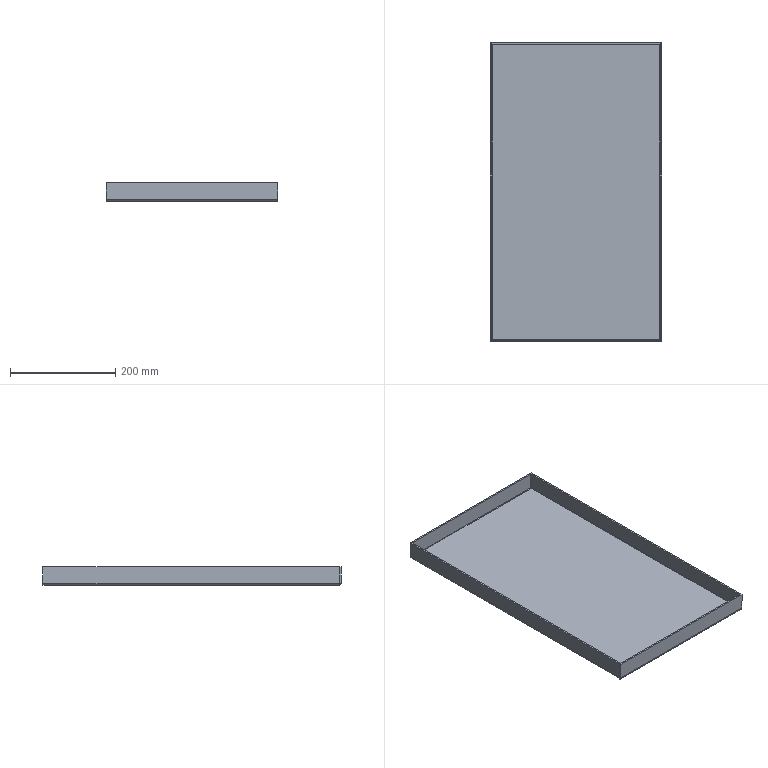Component | SolidWorks | MainBoardLowerBucklePlate-1 | 1 solid | 42 faces | box 326 x 566.5 x 35 mm | volume 718865 mm3 | plane 34 | cylinder 8 | commonest cylinder face diameters 7.473 x4 1.473 x4 | material Q235
STEP:
#1=CARTESIAN_POINT('',(-38.422,4.209,109.595));
#2=VERTEX_POINT('',#1);
#3=CARTESIAN_POINT('',(-38.422,4.206,109.595));
#4=VERTEX_POINT('',#3);
#5=CARTESIAN_POINT('',(-38.422,4.209,109.595));
#6=DIRECTION('',(-0.,-1.,-0.));
#7=VECTOR('',#6,39.37);
#8=LINE('',#5,#7);
#9=EDGE_CURVE('',#2,#4,#8,.T.);
#10=ORIENTED_EDGE('',*,*,#9,.T.);
#11=CARTESIAN_POINT('',(-38.422,4.062,109.477));
#12=VERTEX_POINT('',#11);
#13=CARTESIAN_POINT('',(-38.422,4.062,109.624));
#14=DIRECTION('',(-1.,-0.,0.));
#15=DIRECTION('',(0.,-0.,1.));
#16=AXIS2_PLACEMENT_3D('',#13,#14,#15);
#17=CIRCLE('',#16,0.1471);
#18=EDGE_CURVE('',#4,#12,#17,.T.);
#19=ORIENTED_EDGE('',*,*,#18,.T.);
#20=CARTESIAN_POINT('',(-38.422,4.209,109.477));
#21=VERTEX_POINT('',#20);
#22=CARTESIAN_POINT('',(-38.422,-17.947,109.477));
#23=DIRECTION('',(0.,-1.,-0.));
#24=VECTOR('',#23,39.37);
#25=LINE('',#22,#24);
#26=EDGE_CURVE('',#21,#12,#25,.T.);
#27=ORIENTED_EDGE('',*,*,#26,.F.);
#28=CARTESIAN_POINT('',(-38.422,4.209,109.595));
#29=DIRECTION('',(-0.,0.,-1.));
#30=VECTOR('',#29,39.37);
#31=LINE('',#28,#30);
#32=EDGE_CURVE('',#2,#21,#31,.T.);
#33=ORIENTED_EDGE('',*,*,#32,.F.);
#34=EDGE_LOOP('',(#10,#19,#27,#33));
#35=FACE_OUTER_BOUND('',#34,.T.);
#36=CARTESIAN_POINT('',(-38.422,4.209,109.595));
#37=DIRECTION('',(1.,-0.,-0.));
#38=DIRECTION('',(0.,1.,0.));
#39=AXIS2_PLACEMENT_3D('',#36,#37,#38);
#40=PLANE('',#39);
#41=ADVANCED_FACE('',(#35),#40,.T.);
#42=CARTESIAN_POINT('',(-25.882,4.209,109.477));
#43=VERTEX_POINT('',#42);
#44=CARTESIAN_POINT('',(-25.882,4.062,109.477));
#45=VERTEX_POINT('',#44);
#46=CARTESIAN_POINT('',(-25.882,4.209,109.477));
#47=DIRECTION('',(0.,-1.,-0.));
#48=VECTOR('',#47,39.37);
#49=LINE('',#46,#48);
#50=EDGE_CURVE('',#43,#45,#49,.T.);
#51=ORIENTED_EDGE('',*,*,#50,.T.);
#52=CARTESIAN_POINT('',(-25.882,4.206,109.595));
#53=VERTEX_POINT('',#52);
#54=CARTESIAN_POINT('',(-25.882,4.062,109.624));
#55=DIRECTION('',(1.,0.,-0.));
#56=DIRECTION('',(0.,0.,1.));
#57=AXIS2_PLACEMENT_3D('',#54,#55,#56);
#58=CIRCLE('',#57,0.1471);
#59=EDGE_CURVE('',#45,#53,#58,.T.);
#60=ORIENTED_EDGE('',*,*,#59,.T.);
#61=CARTESIAN_POINT('',(-25.882,4.209,109.595));
#62=VERTEX_POINT('',#61);
#63=CARTESIAN_POINT('',(-25.882,4.209,109.595));
#64=DIRECTION('',(0.,-1.,-0.));
#65=VECTOR('',#64,39.37);
#66=LINE('',#63,#65);
#67=EDGE_CURVE('',#62,#53,#66,.T.);
#68=ORIENTED_EDGE('',*,*,#67,.F.);
#69=CARTESIAN_POINT('',(-25.882,4.209,109.595));
#70=DIRECTION('',(-0.,0.,-1.));
#71=VECTOR('',#70,39.37);
#72=LINE('',#69,#71);
#73=EDGE_CURVE('',#62,#43,#72,.T.);
#74=ORIENTED_EDGE('',*,*,#73,.T.);
#75=EDGE_LOOP('',(#51,#60,#68,#74));
#76=FACE_OUTER_BOUND('',#75,.T.);
#77=CARTESIAN_POINT('',(-25.882,4.062,109.595));
#78=DIRECTION('',(-1.,0.,0.));
#79=DIRECTION('',(-0.,-1.,-0.));
#80=AXIS2_PLACEMENT_3D('',#77,#78,#79);
#81=PLANE('',#80);
#82=ADVANCED_FACE('',(#76),#81,.T.);
#83=CARTESIAN_POINT('',(-38.422,4.062,109.477));
#84=DIRECTION('',(1.,0.,-0.));
#85=VECTOR('',#84,39.37);
#86=LINE('',#83,#85);
#87=EDGE_CURVE('',#12,#45,#86,.T.);
#88=ORIENTED_EDGE('',*,*,#87,.T.);
#89=CARTESIAN_POINT('',(-25.882,-17.947,109.477));
#90=VERTEX_POINT('',#89);
#91=CARTESIAN_POINT('',(-25.882,4.209,109.477));
#92=DIRECTION('',(0.,-1.,-0.));
#93=VECTOR('',#92,39.37);
#94=LINE('',#91,#93);
#95=EDGE_CURVE('',#45,#90,#94,.T.);
#96=ORIENTED_EDGE('',*,*,#95,.T.);
#97=CARTESIAN_POINT('',(-38.422,-17.947,109.477));
#98=VERTEX_POINT('',#97);
#99=CARTESIAN_POINT('',(-25.734,-17.947,109.477));
#100=DIRECTION('',(-1.,-0.,0.));
#101=VECTOR('',#100,39.37);
#102=LINE('',#99,#101);
#103=EDGE_CURVE('',#90,#98,#102,.T.);
#104=ORIENTED_EDGE('',*,*,#103,.T.);
#105=CARTESIAN_POINT('',(-38.422,-17.947,109.477));
#106=DIRECTION('',(-0.,1.,0.));
#107=VECTOR('',#106,39.37);
#108=LINE('',#105,#107);
#109=EDGE_CURVE('',#98,#12,#108,.T.);
#110=ORIENTED_EDGE('',*,*,#109,.T.);
#111=EDGE_LOOP('',(#88,#96,#104,#110));
#112=FACE_OUTER_BOUND('',#111,.T.);
#113=CARTESIAN_POINT('',(-32.152,-6.942,109.477));
#114=DIRECTION('',(0.,-0.,1.));
#115=DIRECTION('',(-0.,1.,0.));
#116=AXIS2_PLACEMENT_3D('',#113,#114,#115);
#117=PLANE('',#116);
#118=ADVANCED_FACE('',(#112),#117,.F.);
#119=CARTESIAN_POINT('',(-25.882,4.062,109.595));
#120=VERTEX_POINT('',#119);
#121=CARTESIAN_POINT('',(-25.882,-17.947,109.595));
#122=VERTEX_POINT('',#121);
#123=CARTESIAN_POINT('',(-25.882,4.209,109.595));
#124=DIRECTION('',(0.,-1.,-0.));
#125=VECTOR('',#124,39.37);
#126=LINE('',#123,#125);
#127=EDGE_CURVE('',#120,#122,#126,.T.);
#128=ORIENTED_EDGE('',*,*,#127,.F.);
#129=CARTESIAN_POINT('',(-38.422,4.062,109.595));
#130=VERTEX_POINT('',#129);
#131=CARTESIAN_POINT('',(-38.422,4.062,109.595));
#132=DIRECTION('',(1.,0.,-0.));
#133=VECTOR('',#132,39.37);
#134=LINE('',#131,#133);
#135=EDGE_CURVE('',#130,#120,#134,.T.);
#136=ORIENTED_EDGE('',*,*,#135,.F.);
#137=CARTESIAN_POINT('',(-38.422,-17.947,109.595));
#138=VERTEX_POINT('',#137);
#139=CARTESIAN_POINT('',(-38.422,-17.947,109.595));
#140=DIRECTION('',(-0.,1.,0.));
#141=VECTOR('',#140,39.37);
#142=LINE('',#139,#141);
#143=EDGE_CURVE('',#138,#130,#142,.T.);
#144=ORIENTED_EDGE('',*,*,#143,.F.);
#145=CARTESIAN_POINT('',(-25.734,-17.947,109.595));
#146=DIRECTION('',(-1.,-0.,0.));
#147=VECTOR('',#146,39.37);
#148=LINE('',#145,#147);
#149=EDGE_CURVE('',#122,#138,#148,.T.);
#150=ORIENTED_EDGE('',*,*,#149,.F.);
#151=EDGE_LOOP('',(#128,#136,#144,#150));
#152=FACE_OUTER_BOUND('',#151,.T.);
#153=CARTESIAN_POINT('',(-32.152,-6.942,109.595));
#154=DIRECTION('',(0.,-0.,1.));
#155=DIRECTION('',(-0.,1.,0.));
#156=AXIS2_PLACEMENT_3D('',#153,#154,#155);
#157=PLANE('',#156);
#158=ADVANCED_FACE('',(#152),#157,.T.);
#159=CARTESIAN_POINT('',(-25.734,-17.947,109.477));
#160=VERTEX_POINT('',#159);
#161=CARTESIAN_POINT('',(-25.734,-17.947,109.477));
#162=DIRECTION('',(-1.,-0.,0.));
#163=VECTOR('',#162,39.37);
#164=LINE('',#161,#163);
#165=EDGE_CURVE('',#160,#90,#164,.T.);
#166=ORIENTED_EDGE('',*,*,#165,.T.);
#167=CARTESIAN_POINT('',(-25.737,-17.947,109.595));
#168=VERTEX_POINT('',#167);
#169=CARTESIAN_POINT('',(-25.882,-17.947,109.624));
#170=DIRECTION('',(0.,-1.,-0.));
#171=DIRECTION('',(0.,0.,-1.));
#172=AXIS2_PLACEMENT_3D('',#169,#170,#171);
#173=CIRCLE('',#172,0.1471);
#174=EDGE_CURVE('',#90,#168,#173,.T.);
#175=ORIENTED_EDGE('',*,*,#174,.T.);
#176=CARTESIAN_POINT('',(-25.734,-17.947,109.595));
#177=VERTEX_POINT('',#176);
#178=CARTESIAN_POINT('',(-25.734,-17.947,109.595));
#179=DIRECTION('',(-1.,-0.,0.));
#180=VECTOR('',#179,39.37);
#181=LINE('',#178,#180);
#182=EDGE_CURVE('',#177,#168,#181,.T.);
#183=ORIENTED_EDGE('',*,*,#182,.F.);
#184=CARTESIAN_POINT('',(-25.734,-17.947,109.595));
#185=DIRECTION('',(-0.,0.,-1.));
#186=VECTOR('',#185,39.37);
#187=LINE('',#184,#186);
#188=EDGE_CURVE('',#177,#160,#187,.T.);
#189=ORIENTED_EDGE('',*,*,#188,.T.);
#190=EDGE_LOOP('',(#166,#175,#183,#189));
#191=FACE_OUTER_BOUND('',#190,.T.);
#192=CARTESIAN_POINT('',(-25.882,-17.947,109.595));
#193=DIRECTION('',(-0.,1.,0.));
#194=DIRECTION('',(-0.,0.,-1.));
#195=AXIS2_PLACEMENT_3D('',#192,#193,#194);
#196=PLANE('',#195);
#197=ADVANCED_FACE('',(#191),#196,.T.);
#198=CARTESIAN_POINT('',(-38.569,-17.947,109.595));
#199=VERTEX_POINT('',#198);
#200=CARTESIAN_POINT('',(-38.566,-17.947,109.595));
#201=VERTEX_POINT('',#200);
#202=CARTESIAN_POINT('',(-38.569,-17.947,109.595));
#203=DIRECTION('',(1.,0.,0.));
#204=VECTOR('',#203,39.37);
#205=LINE('',#202,#204);
#206=EDGE_CURVE('',#199,#201,#205,.T.);
#207=ORIENTED_EDGE('',*,*,#206,.T.);
#208=CARTESIAN_POINT('',(-38.422,-17.947,109.624));
#209=DIRECTION('',(0.,-1.,-0.));
#210=DIRECTION('',(0.,0.,1.));
#211=AXIS2_PLACEMENT_3D('',#208,#209,#210);
#212=CIRCLE('',#211,0.1471);
#213=EDGE_CURVE('',#201,#98,#212,.T.);
#214=ORIENTED_EDGE('',*,*,#213,.T.);
#215=CARTESIAN_POINT('',(-38.569,-17.947,109.477));
#216=VERTEX_POINT('',#215);
#217=CARTESIAN_POINT('',(-25.734,-17.947,109.477));
#218=DIRECTION('',(1.,0.,-0.));
#219=VECTOR('',#218,39.37);
#220=LINE('',#217,#219);
#221=EDGE_CURVE('',#216,#98,#220,.T.);
#222=ORIENTED_EDGE('',*,*,#221,.F.);
#223=CARTESIAN_POINT('',(-38.569,-17.947,109.595));
#224=DIRECTION('',(-0.,0.,-1.));
#225=VECTOR('',#224,39.37);
#226=LINE('',#223,#225);
#227=EDGE_CURVE('',#199,#216,#226,.T.);
#228=ORIENTED_EDGE('',*,*,#227,.F.);
#229=EDGE_LOOP('',(#207,#214,#222,#228));
#230=FACE_OUTER_BOUND('',#229,.T.);
#231=CARTESIAN_POINT('',(-38.569,-17.947,109.595));
#232=DIRECTION('',(-0.,1.,0.));
#233=DIRECTION('',(-0.,0.,-1.));
#234=AXIS2_PLACEMENT_3D('',#231,#232,#233);
#235=PLANE('',#234);
#236=ADVANCED_FACE('',(#230),#235,.T.);
#237=CARTESIAN_POINT('',(-38.569,-17.976,109.624));
#238=VERTEX_POINT('',#237);
#239=CARTESIAN_POINT('',(-38.569,-18.094,109.624));
#240=VERTEX_POINT('',#239);
#241=CARTESIAN_POINT('',(-38.569,-18.094,109.624));
#242=DIRECTION('',(0.,-1.,-0.));
#243=VECTOR('',#242,39.37);
#244=LINE('',#241,#243);
#245=EDGE_CURVE('',#238,#240,#244,.T.);
#246=ORIENTED_EDGE('',*,*,#245,.F.);
#247=CARTESIAN_POINT('',(-38.569,-17.947,109.624));
#248=DIRECTION('',(-1.,-0.,0.));
#249=DIRECTION('',(0.,0.,-1.));
#250=AXIS2_PLACEMENT_3D('',#247,#248,#249);
#251=CIRCLE('',#250,0.029);
#252=EDGE_CURVE('',#199,#238,#251,.T.);
#253=ORIENTED_EDGE('',*,*,#252,.F.);
#254=ORIENTED_EDGE('',*,*,#227,.T.);
#255=CARTESIAN_POINT('',(-38.569,-17.947,109.624));
#256=DIRECTION('',(-1.,-0.,0.));
#257=DIRECTION('',(0.,0.,-1.));
#258=AXIS2_PLACEMENT_3D('',#255,#256,#257);
#259=CIRCLE('',#258,0.1471);
#260=EDGE_CURVE('',#216,#240,#259,.T.);
#261=ORIENTED_EDGE('',*,*,#260,.T.);
#262=EDGE_LOOP('',(#246,#253,#254,#261));
#263=FACE_OUTER_BOUND('',#262,.T.);
#264=CARTESIAN_POINT('',(-38.569,-17.947,109.624));
#265=DIRECTION('',(-1.,-0.,0.));
#266=DIRECTION('',(0.,-0.,1.));
#267=AXIS2_PLACEMENT_3D('',#264,#265,#266);
#268=PLANE('',#267);
#269=ADVANCED_FACE('',(#263),#268,.T.);
#270=CARTESIAN_POINT('',(-25.734,-17.976,109.624));
#271=VERTEX_POINT('',#270);
#272=CARTESIAN_POINT('',(-25.734,-17.947,109.624));
#273=DIRECTION('',(1.,0.,-0.));
#274=DIRECTION('',(0.,0.,-1.));
#275=AXIS2_PLACEMENT_3D('',#272,#273,#274);
#276=CIRCLE('',#275,0.029);
#277=EDGE_CURVE('',#271,#177,#276,.T.);
#278=ORIENTED_EDGE('',*,*,#277,.F.);
#279=CARTESIAN_POINT('',(-25.734,-18.094,109.624));
#280=VERTEX_POINT('',#279);
#281=CARTESIAN_POINT('',(-25.734,-17.976,109.624));
#282=DIRECTION('',(0.,-1.,-0.));
#283=VECTOR('',#282,39.37);
#284=LINE('',#281,#283);
#285=EDGE_CURVE('',#271,#280,#284,.T.);
#286=ORIENTED_EDGE('',*,*,#285,.T.);
#287=CARTESIAN_POINT('',(-25.734,-17.947,109.624));
#288=DIRECTION('',(1.,0.,-0.));
#289=DIRECTION('',(0.,0.,-1.));
#290=AXIS2_PLACEMENT_3D('',#287,#288,#289);
#291=CIRCLE('',#290,0.1471);
#292=EDGE_CURVE('',#280,#160,#291,.T.);
#293=ORIENTED_EDGE('',*,*,#292,.T.);
#294=ORIENTED_EDGE('',*,*,#188,.F.);
#295=EDGE_LOOP('',(#278,#286,#293,#294));
#296=FACE_OUTER_BOUND('',#295,.T.);
#297=CARTESIAN_POINT('',(-25.734,-17.947,109.624));
#298=DIRECTION('',(-1.,-0.,0.));
#299=DIRECTION('',(0.,-0.,1.));
#300=AXIS2_PLACEMENT_3D('',#297,#298,#299);
#301=PLANE('',#300);
#302=ADVANCED_FACE('',(#296),#301,.F.);
#303=ORIENTED_EDGE('',*,*,#165,.F.);
#304=ORIENTED_EDGE('',*,*,#292,.F.);
#305=CARTESIAN_POINT('',(-32.152,-18.094,109.624));
#306=DIRECTION('',(1.,0.,-0.));
#307=VECTOR('',#306,39.37);
#308=LINE('',#305,#307);
#309=EDGE_CURVE('',#240,#280,#308,.T.);
#310=ORIENTED_EDGE('',*,*,#309,.F.);
#311=ORIENTED_EDGE('',*,*,#260,.F.);
#312=ORIENTED_EDGE('',*,*,#221,.T.);
#313=ORIENTED_EDGE('',*,*,#103,.F.);
#314=EDGE_LOOP('',(#303,#304,#310,#311,#312,#313));
#315=FACE_OUTER_BOUND('',#314,.T.);
#316=CARTESIAN_POINT('',(-25.734,-17.947,109.624));
#317=DIRECTION('',(1.,0.,-0.));
#318=DIRECTION('',(0.,-1.,0.));
#319=AXIS2_PLACEMENT_3D('',#316,#317,#318);
#320=CYLINDRICAL_SURFACE('',#319,0.1471);
#321=ADVANCED_FACE('',(#315),#320,.T.);
#322=ORIENTED_EDGE('',*,*,#182,.T.);
#323=CARTESIAN_POINT('',(-25.734,-17.947,109.595));
#324=DIRECTION('',(-1.,-0.,0.));
#325=VECTOR('',#324,39.37);
#326=LINE('',#323,#325);
#327=EDGE_CURVE('',#168,#122,#326,.T.);
#328=ORIENTED_EDGE('',*,*,#327,.T.);
#329=ORIENTED_EDGE('',*,*,#149,.T.);
#330=CARTESIAN_POINT('',(-38.569,-17.947,109.595));
#331=DIRECTION('',(1.,0.,0.));
#332=VECTOR('',#331,39.37);
#333=LINE('',#330,#332);
#334=EDGE_CURVE('',#201,#138,#333,.T.);
#335=ORIENTED_EDGE('',*,*,#334,.F.);
#336=ORIENTED_EDGE('',*,*,#206,.F.);
#337=ORIENTED_EDGE('',*,*,#252,.T.);
#338=CARTESIAN_POINT('',(-38.569,-17.976,109.624));
#339=DIRECTION('',(1.,0.,-0.));
#340=VECTOR('',#339,39.37);
#341=LINE('',#338,#340);
#342=EDGE_CURVE('',#238,#271,#341,.T.);
#343=ORIENTED_EDGE('',*,*,#342,.T.);
#344=ORIENTED_EDGE('',*,*,#277,.T.);
#345=EDGE_LOOP('',(#322,#328,#329,#335,#336,#337,#343,#344));
#346=FACE_OUTER_BOUND('',#345,.T.);
#347=CARTESIAN_POINT('',(-25.734,-17.947,109.624));
#348=DIRECTION('',(1.,0.,-0.));
#349=DIRECTION('',(0.,-1.,0.));
#350=AXIS2_PLACEMENT_3D('',#347,#348,#349);
#351=CYLINDRICAL_SURFACE('',#350,0.029);
#352=ADVANCED_FACE('',(#346),#351,.F.);
#353=CARTESIAN_POINT('',(-25.734,-18.094,110.855));
#354=VERTEX_POINT('',#353);
#355=CARTESIAN_POINT('',(-25.734,-18.094,109.595));
#356=DIRECTION('',(0.,0.,-1.));
#357=VECTOR('',#356,39.37);
#358=LINE('',#355,#357);
#359=EDGE_CURVE('',#354,#280,#358,.T.);
#360=ORIENTED_EDGE('',*,*,#359,.T.);
#361=ORIENTED_EDGE('',*,*,#285,.F.);
#362=CARTESIAN_POINT('',(-25.734,-17.976,110.855));
#363=VERTEX_POINT('',#362);
#364=CARTESIAN_POINT('',(-25.734,-17.976,109.595));
#365=DIRECTION('',(0.,0.,-1.));
#366=VECTOR('',#365,39.37);
#367=LINE('',#364,#366);
#368=EDGE_CURVE('',#363,#271,#367,.T.);
#369=ORIENTED_EDGE('',*,*,#368,.F.);
#370=CARTESIAN_POINT('',(-25.734,-18.094,110.855));
#371=DIRECTION('',(-0.,1.,0.));
#372=VECTOR('',#371,39.37);
#373=LINE('',#370,#372);
#374=EDGE_CURVE('',#354,#363,#373,.T.);
#375=ORIENTED_EDGE('',*,*,#374,.F.);
#376=EDGE_LOOP('',(#360,#361,#369,#375));
#377=FACE_OUTER_BOUND('',#376,.T.);
#378=CARTESIAN_POINT('',(-25.734,-18.094,109.595));
#379=DIRECTION('',(1.,0.,0.));
#380=DIRECTION('',(0.,0.,-1.));
#381=AXIS2_PLACEMENT_3D('',#378,#379,#380);
#382=PLANE('',#381);
#383=ADVANCED_FACE('',(#377),#382,.T.);
#384=CARTESIAN_POINT('',(-38.569,-17.976,110.855));
#385=VERTEX_POINT('',#384);
#386=CARTESIAN_POINT('',(-38.569,-17.976,109.595));
#387=DIRECTION('',(-0.,-0.,1.));
#388=VECTOR('',#387,39.37);
#389=LINE('',#386,#388);
#390=EDGE_CURVE('',#238,#385,#389,.T.);
#391=ORIENTED_EDGE('',*,*,#390,.F.);
#392=ORIENTED_EDGE('',*,*,#245,.T.);
#393=CARTESIAN_POINT('',(-38.569,-18.094,110.855));
#394=VERTEX_POINT('',#393);
#395=CARTESIAN_POINT('',(-38.569,-18.094,110.855));
#396=DIRECTION('',(-0.,-0.,1.));
#397=VECTOR('',#396,39.37);
#398=LINE('',#395,#397);
#399=EDGE_CURVE('',#240,#394,#398,.T.);
#400=ORIENTED_EDGE('',*,*,#399,.T.);
#401=CARTESIAN_POINT('',(-38.569,-18.094,110.855));
#402=DIRECTION('',(-0.,1.,0.));
#403=VECTOR('',#402,39.37);
#404=LINE('',#401,#403);
#405=EDGE_CURVE('',#394,#385,#404,.T.);
#406=ORIENTED_EDGE('',*,*,#405,.T.);
#407=EDGE_LOOP('',(#391,#392,#400,#406));
#408=FACE_OUTER_BOUND('',#407,.T.);
#409=CARTESIAN_POINT('',(-38.569,-18.094,110.855));
#410=DIRECTION('',(-1.,-0.,-0.));
#411=DIRECTION('',(-0.,-0.,1.));
#412=AXIS2_PLACEMENT_3D('',#409,#410,#411);
#413=PLANE('',#412);
#414=ADVANCED_FACE('',(#408),#413,.T.);
#415=ORIENTED_EDGE('',*,*,#399,.F.);
#416=ORIENTED_EDGE('',*,*,#309,.T.);
#417=ORIENTED_EDGE('',*,*,#359,.F.);
#418=CARTESIAN_POINT('',(-25.734,-18.094,110.855));
#419=DIRECTION('',(1.,0.,-0.));
#420=VECTOR('',#419,39.37);
#421=LINE('',#418,#420);
#422=EDGE_CURVE('',#394,#354,#421,.T.);
#423=ORIENTED_EDGE('',*,*,#422,.F.);
#424=EDGE_LOOP('',(#415,#416,#417,#423));
#425=FACE_OUTER_BOUND('',#424,.T.);
#426=CARTESIAN_POINT('',(-32.152,-18.094,109.595));
#427=DIRECTION('',(0.,-1.,-0.));
#428=DIRECTION('',(0.,-0.,1.));
#429=AXIS2_PLACEMENT_3D('',#426,#427,#428);
#430=PLANE('',#429);
#431=ADVANCED_FACE('',(#425),#430,.T.);
#432=ORIENTED_EDGE('',*,*,#342,.F.);
#433=ORIENTED_EDGE('',*,*,#390,.T.);
#434=CARTESIAN_POINT('',(-32.152,-17.976,110.855));
#435=DIRECTION('',(1.,0.,-0.));
#436=VECTOR('',#435,39.37);
#437=LINE('',#434,#436);
#438=EDGE_CURVE('',#385,#363,#437,.T.);
#439=ORIENTED_EDGE('',*,*,#438,.T.);
#440=ORIENTED_EDGE('',*,*,#368,.T.);
#441=EDGE_LOOP('',(#432,#433,#439,#440));
#442=FACE_OUTER_BOUND('',#441,.T.);
#443=CARTESIAN_POINT('',(-32.152,-17.976,109.595));
#444=DIRECTION('',(0.,-1.,-0.));
#445=DIRECTION('',(0.,-0.,1.));
#446=AXIS2_PLACEMENT_3D('',#443,#444,#445);
#447=PLANE('',#446);
#448=ADVANCED_FACE('',(#442),#447,.F.);
#449=ORIENTED_EDGE('',*,*,#438,.F.);
#450=ORIENTED_EDGE('',*,*,#405,.F.);
#451=ORIENTED_EDGE('',*,*,#422,.T.);
#452=ORIENTED_EDGE('',*,*,#374,.T.);
#453=EDGE_LOOP('',(#449,#450,#451,#452));
#454=FACE_OUTER_BOUND('',#453,.T.);
#455=CARTESIAN_POINT('',(-25.734,-18.094,110.855));
#456=DIRECTION('',(0.,-0.,1.));
#457=DIRECTION('',(-0.,1.,0.));
#458=AXIS2_PLACEMENT_3D('',#455,#456,#457);
#459=PLANE('',#458);
#460=ADVANCED_FACE('',(#454),#459,.T.);
#461=CARTESIAN_POINT('',(-38.451,4.209,109.624));
#462=VERTEX_POINT('',#461);
#463=CARTESIAN_POINT('',(-38.569,4.209,109.624));
#464=VERTEX_POINT('',#463);
#465=CARTESIAN_POINT('',(-38.569,4.209,109.624));
#466=DIRECTION('',(-1.,-0.,-0.));
#467=VECTOR('',#466,39.37);
#468=LINE('',#465,#467);
#469=EDGE_CURVE('',#462,#464,#468,.T.);
#470=ORIENTED_EDGE('',*,*,#469,.F.);
#471=CARTESIAN_POINT('',(-38.422,4.209,109.624));
#472=DIRECTION('',(-0.,1.,0.));
#473=DIRECTION('',(0.,0.,1.));
#474=AXIS2_PLACEMENT_3D('',#471,#472,#473);
#475=CIRCLE('',#474,0.029);
#476=EDGE_CURVE('',#2,#462,#475,.T.);
#477=ORIENTED_EDGE('',*,*,#476,.F.);
#478=ORIENTED_EDGE('',*,*,#32,.T.);
#479=CARTESIAN_POINT('',(-38.422,4.209,109.624));
#480=DIRECTION('',(-0.,1.,0.));
#481=DIRECTION('',(0.,-0.,1.));
#482=AXIS2_PLACEMENT_3D('',#479,#480,#481);
#483=CIRCLE('',#482,0.1471);
#484=EDGE_CURVE('',#21,#464,#483,.T.);
#485=ORIENTED_EDGE('',*,*,#484,.T.);
#486=EDGE_LOOP('',(#470,#477,#478,#485));
#487=FACE_OUTER_BOUND('',#486,.T.);
#488=CARTESIAN_POINT('',(-38.422,4.209,109.624));
#489=DIRECTION('',(-0.,1.,0.));
#490=DIRECTION('',(-0.,0.,-1.));
#491=AXIS2_PLACEMENT_3D('',#488,#489,#490);
#492=PLANE('',#491);
#493=ADVANCED_FACE('',(#487),#492,.T.);
#494=CARTESIAN_POINT('',(-38.569,-17.947,109.624));
#495=VERTEX_POINT('',#494);
#496=CARTESIAN_POINT('',(-38.422,-17.947,109.624));
#497=DIRECTION('',(0.,-1.,-0.));
#498=DIRECTION('',(0.,0.,1.));
#499=AXIS2_PLACEMENT_3D('',#496,#497,#498);
#500=CIRCLE('',#499,0.1471);
#501=EDGE_CURVE('',#495,#201,#500,.T.);
#502=ORIENTED_EDGE('',*,*,#501,.T.);
#503=ORIENTED_EDGE('',*,*,#334,.T.);
#504=CARTESIAN_POINT('',(-38.451,-17.947,109.624));
#505=VERTEX_POINT('',#504);
#506=CARTESIAN_POINT('',(-38.422,-17.947,109.624));
#507=DIRECTION('',(0.,-1.,-0.));
#508=DIRECTION('',(0.,0.,1.));
#509=AXIS2_PLACEMENT_3D('',#506,#507,#508);
#510=CIRCLE('',#509,0.029);
#511=EDGE_CURVE('',#505,#138,#510,.T.);
#512=ORIENTED_EDGE('',*,*,#511,.F.);
#513=CARTESIAN_POINT('',(-38.451,-17.947,109.624));
#514=DIRECTION('',(-1.,-0.,-0.));
#515=VECTOR('',#514,39.37);
#516=LINE('',#513,#515);
#517=EDGE_CURVE('',#505,#495,#516,.T.);
#518=ORIENTED_EDGE('',*,*,#517,.T.);
#519=EDGE_LOOP('',(#502,#503,#512,#518));
#520=FACE_OUTER_BOUND('',#519,.T.);
#521=CARTESIAN_POINT('',(-38.422,-17.947,109.624));
#522=DIRECTION('',(-0.,1.,0.));
#523=DIRECTION('',(-0.,0.,-1.));
#524=AXIS2_PLACEMENT_3D('',#521,#522,#523);
#525=PLANE('',#524);
#526=ADVANCED_FACE('',(#520),#525,.F.);
#527=ORIENTED_EDGE('',*,*,#109,.F.);
#528=ORIENTED_EDGE('',*,*,#213,.F.);
#529=ORIENTED_EDGE('',*,*,#501,.F.);
#530=CARTESIAN_POINT('',(-38.569,-6.942,109.624));
#531=DIRECTION('',(0.,-1.,-0.));
#532=VECTOR('',#531,39.37);
#533=LINE('',#530,#532);
#534=EDGE_CURVE('',#464,#495,#533,.T.);
#535=ORIENTED_EDGE('',*,*,#534,.F.);
#536=ORIENTED_EDGE('',*,*,#484,.F.);
#537=ORIENTED_EDGE('',*,*,#26,.T.);
#538=EDGE_LOOP('',(#527,#528,#529,#535,#536,#537));
#539=FACE_OUTER_BOUND('',#538,.T.);
#540=CARTESIAN_POINT('',(-38.422,-17.947,109.624));
#541=DIRECTION('',(0.,-1.,-0.));
#542=DIRECTION('',(-1.,0.,0.));
#543=AXIS2_PLACEMENT_3D('',#540,#541,#542);
#544=CYLINDRICAL_SURFACE('',#543,0.1471);
#545=ADVANCED_FACE('',(#539),#544,.T.);
#546=ORIENTED_EDGE('',*,*,#143,.T.);
#547=CARTESIAN_POINT('',(-38.422,4.209,109.595));
#548=DIRECTION('',(-0.,-1.,-0.));
#549=VECTOR('',#548,39.37);
#550=LINE('',#547,#549);
#551=EDGE_CURVE('',#4,#130,#550,.T.);
#552=ORIENTED_EDGE('',*,*,#551,.F.);
#553=ORIENTED_EDGE('',*,*,#9,.F.);
#554=ORIENTED_EDGE('',*,*,#476,.T.);
#555=CARTESIAN_POINT('',(-38.451,4.209,109.624));
#556=DIRECTION('',(0.,-1.,-0.));
#557=VECTOR('',#556,39.37);
#558=LINE('',#555,#557);
#559=EDGE_CURVE('',#462,#505,#558,.T.);
#560=ORIENTED_EDGE('',*,*,#559,.T.);
#561=ORIENTED_EDGE('',*,*,#511,.T.);
#562=EDGE_LOOP('',(#546,#552,#553,#554,#560,#561));
#563=FACE_OUTER_BOUND('',#562,.T.);
#564=CARTESIAN_POINT('',(-38.422,-17.947,109.624));
#565=DIRECTION('',(0.,-1.,-0.));
#566=DIRECTION('',(-1.,0.,0.));
#567=AXIS2_PLACEMENT_3D('',#564,#565,#566);
#568=CYLINDRICAL_SURFACE('',#567,0.029);
#569=ADVANCED_FACE('',(#563),#568,.F.);
#570=CARTESIAN_POINT('',(-38.569,-17.947,110.855));
#571=VERTEX_POINT('',#570);
#572=CARTESIAN_POINT('',(-38.569,-17.947,109.595));
#573=DIRECTION('',(0.,0.,-1.));
#574=VECTOR('',#573,39.37);
#575=LINE('',#572,#574);
#576=EDGE_CURVE('',#571,#495,#575,.T.);
#577=ORIENTED_EDGE('',*,*,#576,.T.);
#578=ORIENTED_EDGE('',*,*,#517,.F.);
#579=CARTESIAN_POINT('',(-38.451,-17.947,110.855));
#580=VERTEX_POINT('',#579);
#581=CARTESIAN_POINT('',(-38.451,-17.947,109.595));
#582=DIRECTION('',(0.,0.,-1.));
#583=VECTOR('',#582,39.37);
#584=LINE('',#581,#583);
#585=EDGE_CURVE('',#580,#505,#584,.T.);
#586=ORIENTED_EDGE('',*,*,#585,.F.);
#587=CARTESIAN_POINT('',(-38.569,-17.947,110.855));
#588=DIRECTION('',(1.,0.,0.));
#589=VECTOR('',#588,39.37);
#590=LINE('',#587,#589);
#591=EDGE_CURVE('',#571,#580,#590,.T.);
#592=ORIENTED_EDGE('',*,*,#591,.F.);
#593=EDGE_LOOP('',(#577,#578,#586,#592));
#594=FACE_OUTER_BOUND('',#593,.T.);
#595=CARTESIAN_POINT('',(-38.569,-17.947,109.595));
#596=DIRECTION('',(0.,-1.,-0.));
#597=DIRECTION('',(1.,0.,-0.));
#598=AXIS2_PLACEMENT_3D('',#595,#596,#597);
#599=PLANE('',#598);
#600=ADVANCED_FACE('',(#594),#599,.T.);
#601=CARTESIAN_POINT('',(-38.451,4.209,110.855));
#602=VERTEX_POINT('',#601);
#603=CARTESIAN_POINT('',(-38.451,4.209,109.595));
#604=DIRECTION('',(-0.,-0.,1.));
#605=VECTOR('',#604,39.37);
#606=LINE('',#603,#605);
#607=EDGE_CURVE('',#462,#602,#606,.T.);
#608=ORIENTED_EDGE('',*,*,#607,.F.);
#609=ORIENTED_EDGE('',*,*,#469,.T.);
#610=CARTESIAN_POINT('',(-38.569,4.209,110.855));
#611=VERTEX_POINT('',#610);
#612=CARTESIAN_POINT('',(-38.569,4.209,110.855));
#613=DIRECTION('',(-0.,-0.,1.));
#614=VECTOR('',#613,39.37);
#615=LINE('',#612,#614);
#616=EDGE_CURVE('',#464,#611,#615,.T.);
#617=ORIENTED_EDGE('',*,*,#616,.T.);
#618=CARTESIAN_POINT('',(-38.569,4.209,110.855));
#619=DIRECTION('',(1.,0.,0.));
#620=VECTOR('',#619,39.37);
#621=LINE('',#618,#620);
#622=EDGE_CURVE('',#611,#602,#621,.T.);
#623=ORIENTED_EDGE('',*,*,#622,.T.);
#624=EDGE_LOOP('',(#608,#609,#617,#623));
#625=FACE_OUTER_BOUND('',#624,.T.);
#626=CARTESIAN_POINT('',(-38.569,4.209,110.855));
#627=DIRECTION('',(-0.,1.,0.));
#628=DIRECTION('',(-1.,-0.,0.));
#629=AXIS2_PLACEMENT_3D('',#626,#627,#628);
#630=PLANE('',#629);
#631=ADVANCED_FACE('',(#625),#630,.T.);
#632=ORIENTED_EDGE('',*,*,#616,.F.);
#633=ORIENTED_EDGE('',*,*,#534,.T.);
#634=ORIENTED_EDGE('',*,*,#576,.F.);
#635=CARTESIAN_POINT('',(-38.569,-17.947,110.855));
#636=DIRECTION('',(0.,-1.,-0.));
#637=VECTOR('',#636,39.37);
#638=LINE('',#635,#637);
#639=EDGE_CURVE('',#611,#571,#638,.T.);
#640=ORIENTED_EDGE('',*,*,#639,.F.);
#641=EDGE_LOOP('',(#632,#633,#634,#640));
#642=FACE_OUTER_BOUND('',#641,.T.);
#643=CARTESIAN_POINT('',(-38.569,-6.942,109.595));
#644=DIRECTION('',(-1.,-0.,-0.));
#645=DIRECTION('',(-0.,-0.,1.));
#646=AXIS2_PLACEMENT_3D('',#643,#644,#645);
#647=PLANE('',#646);
#648=ADVANCED_FACE('',(#642),#647,.T.);
#649=ORIENTED_EDGE('',*,*,#559,.F.);
#650=ORIENTED_EDGE('',*,*,#607,.T.);
#651=CARTESIAN_POINT('',(-38.451,-6.942,110.855));
#652=DIRECTION('',(0.,-1.,-0.));
#653=VECTOR('',#652,39.37);
#654=LINE('',#651,#653);
#655=EDGE_CURVE('',#602,#580,#654,.T.);
#656=ORIENTED_EDGE('',*,*,#655,.T.);
#657=ORIENTED_EDGE('',*,*,#585,.T.);
#658=EDGE_LOOP('',(#649,#650,#656,#657));
#659=FACE_OUTER_BOUND('',#658,.T.);
#660=CARTESIAN_POINT('',(-38.451,-6.942,109.595));
#661=DIRECTION('',(-1.,-0.,-0.));
#662=DIRECTION('',(-0.,-0.,1.));
#663=AXIS2_PLACEMENT_3D('',#660,#661,#662);
#664=PLANE('',#663);
#665=ADVANCED_FACE('',(#659),#664,.F.);
#666=ORIENTED_EDGE('',*,*,#655,.F.);
#667=ORIENTED_EDGE('',*,*,#622,.F.);
#668=ORIENTED_EDGE('',*,*,#639,.T.);
#669=ORIENTED_EDGE('',*,*,#591,.T.);
#670=EDGE_LOOP('',(#666,#667,#668,#669));
#671=FACE_OUTER_BOUND('',#670,.T.);
#672=CARTESIAN_POINT('',(-38.569,-17.947,110.855));
#673=DIRECTION('',(-0.,-0.,1.));
#674=DIRECTION('',(1.,0.,0.));
#675=AXIS2_PLACEMENT_3D('',#672,#673,#674);
#676=PLANE('',#675);
#677=ADVANCED_FACE('',(#671),#676,.T.);
#678=ORIENTED_EDGE('',*,*,#327,.F.);
#679=CARTESIAN_POINT('',(-25.734,-17.947,109.624));
#680=VERTEX_POINT('',#679);
#681=CARTESIAN_POINT('',(-25.882,-17.947,109.624));
#682=DIRECTION('',(0.,-1.,-0.));
#683=DIRECTION('',(-0.,0.,-1.));
#684=AXIS2_PLACEMENT_3D('',#681,#682,#683);
#685=CIRCLE('',#684,0.1471);
#686=EDGE_CURVE('',#168,#680,#685,.T.);
#687=ORIENTED_EDGE('',*,*,#686,.T.);
#688=CARTESIAN_POINT('',(-25.853,-17.947,109.624));
#689=VERTEX_POINT('',#688);
#690=CARTESIAN_POINT('',(-25.734,-17.947,109.624));
#691=DIRECTION('',(1.,0.,-0.));
#692=VECTOR('',#691,39.37);
#693=LINE('',#690,#692);
#694=EDGE_CURVE('',#689,#680,#693,.T.);
#695=ORIENTED_EDGE('',*,*,#694,.F.);
#696=CARTESIAN_POINT('',(-25.882,-17.947,109.624));
#697=DIRECTION('',(0.,-1.,-0.));
#698=DIRECTION('',(0.,0.,-1.));
#699=AXIS2_PLACEMENT_3D('',#696,#697,#698);
#700=CIRCLE('',#699,0.029);
#701=EDGE_CURVE('',#122,#689,#700,.T.);
#702=ORIENTED_EDGE('',*,*,#701,.F.);
#703=EDGE_LOOP('',(#678,#687,#695,#702));
#704=FACE_OUTER_BOUND('',#703,.T.);
#705=CARTESIAN_POINT('',(-25.882,-17.947,109.624));
#706=DIRECTION('',(0.,-1.,-0.));
#707=DIRECTION('',(0.,-0.,1.));
#708=AXIS2_PLACEMENT_3D('',#705,#706,#707);
#709=PLANE('',#708);
#710=ADVANCED_FACE('',(#704),#709,.T.);
#711=CARTESIAN_POINT('',(-25.853,4.209,109.624));
#712=VERTEX_POINT('',#711);
#713=CARTESIAN_POINT('',(-25.882,4.209,109.624));
#714=DIRECTION('',(-0.,1.,0.));
#715=DIRECTION('',(0.,0.,-1.));
#716=AXIS2_PLACEMENT_3D('',#713,#714,#715);
#717=CIRCLE('',#716,0.029);
#718=EDGE_CURVE('',#712,#62,#717,.T.);
#719=ORIENTED_EDGE('',*,*,#718,.F.);
#720=CARTESIAN_POINT('',(-25.734,4.209,109.624));
#721=VERTEX_POINT('',#720);
#722=CARTESIAN_POINT('',(-25.853,4.209,109.624));
#723=DIRECTION('',(1.,0.,-0.));
#724=VECTOR('',#723,39.37);
#725=LINE('',#722,#724);
#726=EDGE_CURVE('',#712,#721,#725,.T.);
#727=ORIENTED_EDGE('',*,*,#726,.T.);
#728=CARTESIAN_POINT('',(-25.882,4.209,109.624));
#729=DIRECTION('',(-0.,1.,0.));
#730=DIRECTION('',(0.,0.,-1.));
#731=AXIS2_PLACEMENT_3D('',#728,#729,#730);
#732=CIRCLE('',#731,0.1471);
#733=EDGE_CURVE('',#721,#43,#732,.T.);
#734=ORIENTED_EDGE('',*,*,#733,.T.);
#735=ORIENTED_EDGE('',*,*,#73,.F.);
#736=EDGE_LOOP('',(#719,#727,#734,#735));
#737=FACE_OUTER_BOUND('',#736,.T.);
#738=CARTESIAN_POINT('',(-25.882,4.209,109.624));
#739=DIRECTION('',(0.,-1.,-0.));
#740=DIRECTION('',(0.,-0.,1.));
#741=AXIS2_PLACEMENT_3D('',#738,#739,#740);
#742=PLANE('',#741);
#743=ADVANCED_FACE('',(#737),#742,.F.);
#744=ORIENTED_EDGE('',*,*,#50,.F.);
#745=ORIENTED_EDGE('',*,*,#733,.F.);
#746=CARTESIAN_POINT('',(-25.734,-6.942,109.624));
#747=DIRECTION('',(-0.,1.,0.));
#748=VECTOR('',#747,39.37);
#749=LINE('',#746,#748);
#750=EDGE_CURVE('',#680,#721,#749,.T.);
#751=ORIENTED_EDGE('',*,*,#750,.F.);
#752=ORIENTED_EDGE('',*,*,#686,.F.);
#753=ORIENTED_EDGE('',*,*,#174,.F.);
#754=ORIENTED_EDGE('',*,*,#95,.F.);
#755=EDGE_LOOP('',(#744,#745,#751,#752,#753,#754));
#756=FACE_OUTER_BOUND('',#755,.T.);
#757=CARTESIAN_POINT('',(-25.882,4.209,109.624));
#758=DIRECTION('',(-0.,1.,0.));
#759=DIRECTION('',(1.,0.,0.));
#760=AXIS2_PLACEMENT_3D('',#757,#758,#759);
#761=CYLINDRICAL_SURFACE('',#760,0.1471);
#762=ADVANCED_FACE('',(#756),#761,.T.);
#763=ORIENTED_EDGE('',*,*,#67,.T.);
#764=CARTESIAN_POINT('',(-25.882,4.209,109.595));
#765=DIRECTION('',(0.,-1.,-0.));
#766=VECTOR('',#765,39.37);
#767=LINE('',#764,#766);
#768=EDGE_CURVE('',#53,#120,#767,.T.);
#769=ORIENTED_EDGE('',*,*,#768,.T.);
#770=ORIENTED_EDGE('',*,*,#127,.T.);
#771=ORIENTED_EDGE('',*,*,#701,.T.);
#772=CARTESIAN_POINT('',(-25.853,-17.947,109.624));
#773=DIRECTION('',(-0.,1.,0.));
#774=VECTOR('',#773,39.37);
#775=LINE('',#772,#774);
#776=EDGE_CURVE('',#689,#712,#775,.T.);
#777=ORIENTED_EDGE('',*,*,#776,.T.);
#778=ORIENTED_EDGE('',*,*,#718,.T.);
#779=EDGE_LOOP('',(#763,#769,#770,#771,#777,#778));
#780=FACE_OUTER_BOUND('',#779,.T.);
#781=CARTESIAN_POINT('',(-25.882,4.209,109.624));
#782=DIRECTION('',(-0.,1.,0.));
#783=DIRECTION('',(1.,0.,0.));
#784=AXIS2_PLACEMENT_3D('',#781,#782,#783);
#785=CYLINDRICAL_SURFACE('',#784,0.029);
#786=ADVANCED_FACE('',(#780),#785,.F.);
#787=CARTESIAN_POINT('',(-25.734,4.209,110.855));
#788=VERTEX_POINT('',#787);
#789=CARTESIAN_POINT('',(-25.734,4.209,109.595));
#790=DIRECTION('',(-0.,0.,-1.));
#791=VECTOR('',#790,39.37);
#792=LINE('',#789,#791);
#793=EDGE_CURVE('',#788,#721,#792,.T.);
#794=ORIENTED_EDGE('',*,*,#793,.T.);
#795=ORIENTED_EDGE('',*,*,#726,.F.);
#796=CARTESIAN_POINT('',(-25.853,4.209,110.855));
#797=VERTEX_POINT('',#796);
#798=CARTESIAN_POINT('',(-25.853,4.209,109.595));
#799=DIRECTION('',(-0.,0.,-1.));
#800=VECTOR('',#799,39.37);
#801=LINE('',#798,#800);
#802=EDGE_CURVE('',#797,#712,#801,.T.);
#803=ORIENTED_EDGE('',*,*,#802,.F.);
#804=CARTESIAN_POINT('',(-25.734,4.209,110.855));
#805=DIRECTION('',(-1.,-0.,0.));
#806=VECTOR('',#805,39.37);
#807=LINE('',#804,#806);
#808=EDGE_CURVE('',#788,#797,#807,.T.);
#809=ORIENTED_EDGE('',*,*,#808,.F.);
#810=EDGE_LOOP('',(#794,#795,#803,#809));
#811=FACE_OUTER_BOUND('',#810,.T.);
#812=CARTESIAN_POINT('',(-25.734,4.209,109.595));
#813=DIRECTION('',(-0.,1.,0.));
#814=DIRECTION('',(-0.,0.,-1.));
#815=AXIS2_PLACEMENT_3D('',#812,#813,#814);
#816=PLANE('',#815);
#817=ADVANCED_FACE('',(#811),#816,.T.);
#818=CARTESIAN_POINT('',(-25.853,-17.947,110.855));
#819=VERTEX_POINT('',#818);
#820=CARTESIAN_POINT('',(-25.853,-17.947,109.595));
#821=DIRECTION('',(0.,-0.,1.));
#822=VECTOR('',#821,39.37);
#823=LINE('',#820,#822);
#824=EDGE_CURVE('',#689,#819,#823,.T.);
#825=ORIENTED_EDGE('',*,*,#824,.F.);
#826=ORIENTED_EDGE('',*,*,#694,.T.);
#827=CARTESIAN_POINT('',(-25.734,-17.947,110.855));
#828=VERTEX_POINT('',#827);
#829=CARTESIAN_POINT('',(-25.734,-17.947,110.855));
#830=DIRECTION('',(0.,-0.,1.));
#831=VECTOR('',#830,39.37);
#832=LINE('',#829,#831);
#833=EDGE_CURVE('',#680,#828,#832,.T.);
#834=ORIENTED_EDGE('',*,*,#833,.T.);
#835=CARTESIAN_POINT('',(-25.734,-17.947,110.855));
#836=DIRECTION('',(-1.,-0.,0.));
#837=VECTOR('',#836,39.37);
#838=LINE('',#835,#837);
#839=EDGE_CURVE('',#828,#819,#838,.T.);
#840=ORIENTED_EDGE('',*,*,#839,.T.);
#841=EDGE_LOOP('',(#825,#826,#834,#840));
#842=FACE_OUTER_BOUND('',#841,.T.);
#843=CARTESIAN_POINT('',(-25.734,-17.947,110.855));
#844=DIRECTION('',(0.,-1.,-0.));
#845=DIRECTION('',(0.,-0.,1.));
#846=AXIS2_PLACEMENT_3D('',#843,#844,#845);
#847=PLANE('',#846);
#848=ADVANCED_FACE('',(#842),#847,.T.);
#849=ORIENTED_EDGE('',*,*,#833,.F.);
#850=ORIENTED_EDGE('',*,*,#750,.T.);
#851=ORIENTED_EDGE('',*,*,#793,.F.);
#852=CARTESIAN_POINT('',(-25.734,4.209,110.855));
#853=DIRECTION('',(-0.,1.,0.));
#854=VECTOR('',#853,39.37);
#855=LINE('',#852,#854);
#856=EDGE_CURVE('',#828,#788,#855,.T.);
#857=ORIENTED_EDGE('',*,*,#856,.F.);
#858=EDGE_LOOP('',(#849,#850,#851,#857));
#859=FACE_OUTER_BOUND('',#858,.T.);
#860=CARTESIAN_POINT('',(-25.734,-6.942,109.595));
#861=DIRECTION('',(1.,0.,-0.));
#862=DIRECTION('',(-0.,0.,-1.));
#863=AXIS2_PLACEMENT_3D('',#860,#861,#862);
#864=PLANE('',#863);
#865=ADVANCED_FACE('',(#859),#864,.T.);
#866=ORIENTED_EDGE('',*,*,#776,.F.);
#867=ORIENTED_EDGE('',*,*,#824,.T.);
#868=CARTESIAN_POINT('',(-25.853,-6.942,110.855));
#869=DIRECTION('',(-0.,1.,0.));
#870=VECTOR('',#869,39.37);
#871=LINE('',#868,#870);
#872=EDGE_CURVE('',#819,#797,#871,.T.);
#873=ORIENTED_EDGE('',*,*,#872,.T.);
#874=ORIENTED_EDGE('',*,*,#802,.T.);
#875=EDGE_LOOP('',(#866,#867,#873,#874));
#876=FACE_OUTER_BOUND('',#875,.T.);
#877=CARTESIAN_POINT('',(-25.853,-6.942,109.595));
#878=DIRECTION('',(1.,0.,-0.));
#879=DIRECTION('',(-0.,0.,-1.));
#880=AXIS2_PLACEMENT_3D('',#877,#878,#879);
#881=PLANE('',#880);
#882=ADVANCED_FACE('',(#876),#881,.F.);
#883=ORIENTED_EDGE('',*,*,#872,.F.);
#884=ORIENTED_EDGE('',*,*,#839,.F.);
#885=ORIENTED_EDGE('',*,*,#856,.T.);
#886=ORIENTED_EDGE('',*,*,#808,.T.);
#887=EDGE_LOOP('',(#883,#884,#885,#886));
#888=FACE_OUTER_BOUND('',#887,.T.);
#889=CARTESIAN_POINT('',(-25.734,4.209,110.855));
#890=DIRECTION('',(0.,-0.,1.));
#891=DIRECTION('',(1.,0.,-0.));
#892=AXIS2_PLACEMENT_3D('',#889,#890,#891);
#893=PLANE('',#892);
#894=ADVANCED_FACE('',(#888),#893,.T.);
#895=ORIENTED_EDGE('',*,*,#768,.F.);
#896=CARTESIAN_POINT('',(-25.882,4.209,109.624));
#897=VERTEX_POINT('',#896);
#898=CARTESIAN_POINT('',(-25.882,4.062,109.624));
#899=DIRECTION('',(1.,0.,-0.));
#900=DIRECTION('',(0.,-0.,1.));
#901=AXIS2_PLACEMENT_3D('',#898,#899,#900);
#902=CIRCLE('',#901,0.1471);
#903=EDGE_CURVE('',#53,#897,#902,.T.);
#904=ORIENTED_EDGE('',*,*,#903,.T.);
#905=CARTESIAN_POINT('',(-25.882,4.091,109.624));
#906=VERTEX_POINT('',#905);
#907=CARTESIAN_POINT('',(-25.882,4.209,109.624));
#908=DIRECTION('',(-0.,1.,-0.));
#909=VECTOR('',#908,39.37);
#910=LINE('',#907,#909);
#911=EDGE_CURVE('',#906,#897,#910,.T.);
#912=ORIENTED_EDGE('',*,*,#911,.F.);
#913=CARTESIAN_POINT('',(-25.882,4.062,109.624));
#914=DIRECTION('',(1.,0.,-0.));
#915=DIRECTION('',(0.,0.,1.));
#916=AXIS2_PLACEMENT_3D('',#913,#914,#915);
#917=CIRCLE('',#916,0.029);
#918=EDGE_CURVE('',#120,#906,#917,.T.);
#919=ORIENTED_EDGE('',*,*,#918,.F.);
#920=EDGE_LOOP('',(#895,#904,#912,#919));
#921=FACE_OUTER_BOUND('',#920,.T.);
#922=CARTESIAN_POINT('',(-25.882,4.062,109.624));
#923=DIRECTION('',(1.,0.,-0.));
#924=DIRECTION('',(-0.,0.,-1.));
#925=AXIS2_PLACEMENT_3D('',#922,#923,#924);
#926=PLANE('',#925);
#927=ADVANCED_FACE('',(#921),#926,.T.);
#928=CARTESIAN_POINT('',(-38.422,4.209,109.624));
#929=VERTEX_POINT('',#928);
#930=CARTESIAN_POINT('',(-38.422,4.062,109.624));
#931=DIRECTION('',(-1.,-0.,0.));
#932=DIRECTION('',(0.,-0.,1.));
#933=AXIS2_PLACEMENT_3D('',#930,#931,#932);
#934=CIRCLE('',#933,0.1471);
#935=EDGE_CURVE('',#929,#4,#934,.T.);
#936=ORIENTED_EDGE('',*,*,#935,.T.);
#937=ORIENTED_EDGE('',*,*,#551,.T.);
#938=CARTESIAN_POINT('',(-38.422,4.091,109.624));
#939=VERTEX_POINT('',#938);
#940=CARTESIAN_POINT('',(-38.422,4.062,109.624));
#941=DIRECTION('',(-1.,-0.,0.));
#942=DIRECTION('',(0.,0.,1.));
#943=AXIS2_PLACEMENT_3D('',#940,#941,#942);
#944=CIRCLE('',#943,0.029);
#945=EDGE_CURVE('',#939,#130,#944,.T.);
#946=ORIENTED_EDGE('',*,*,#945,.F.);
#947=CARTESIAN_POINT('',(-38.422,4.091,109.624));
#948=DIRECTION('',(-0.,1.,-0.));
#949=VECTOR('',#948,39.37);
#950=LINE('',#947,#949);
#951=EDGE_CURVE('',#939,#929,#950,.T.);
#952=ORIENTED_EDGE('',*,*,#951,.T.);
#953=EDGE_LOOP('',(#936,#937,#946,#952));
#954=FACE_OUTER_BOUND('',#953,.T.);
#955=CARTESIAN_POINT('',(-38.422,4.062,109.624));
#956=DIRECTION('',(1.,0.,-0.));
#957=DIRECTION('',(-0.,0.,-1.));
#958=AXIS2_PLACEMENT_3D('',#955,#956,#957);
#959=PLANE('',#958);
#960=ADVANCED_FACE('',(#954),#959,.F.);
#961=ORIENTED_EDGE('',*,*,#87,.F.);
#962=ORIENTED_EDGE('',*,*,#18,.F.);
#963=ORIENTED_EDGE('',*,*,#935,.F.);
#964=CARTESIAN_POINT('',(-32.152,4.209,109.624));
#965=DIRECTION('',(-1.,-0.,0.));
#966=VECTOR('',#965,39.37);
#967=LINE('',#964,#966);
#968=EDGE_CURVE('',#897,#929,#967,.T.);
#969=ORIENTED_EDGE('',*,*,#968,.F.);
#970=ORIENTED_EDGE('',*,*,#903,.F.);
#971=ORIENTED_EDGE('',*,*,#59,.F.);
#972=EDGE_LOOP('',(#961,#962,#963,#969,#970,#971));
#973=FACE_OUTER_BOUND('',#972,.T.);
#974=CARTESIAN_POINT('',(-38.422,4.062,109.624));
#975=DIRECTION('',(-1.,-0.,0.));
#976=DIRECTION('',(0.,1.,0.));
#977=AXIS2_PLACEMENT_3D('',#974,#975,#976);
#978=CYLINDRICAL_SURFACE('',#977,0.1471);
#979=ADVANCED_FACE('',(#973),#978,.T.);
#980=ORIENTED_EDGE('',*,*,#135,.T.);
#981=ORIENTED_EDGE('',*,*,#918,.T.);
#982=CARTESIAN_POINT('',(-25.882,4.091,109.624));
#983=DIRECTION('',(-1.,-0.,0.));
#984=VECTOR('',#983,39.37);
#985=LINE('',#982,#984);
#986=EDGE_CURVE('',#906,#939,#985,.T.);
#987=ORIENTED_EDGE('',*,*,#986,.T.);
#988=ORIENTED_EDGE('',*,*,#945,.T.);
#989=EDGE_LOOP('',(#980,#981,#987,#988));
#990=FACE_OUTER_BOUND('',#989,.T.);
#991=CARTESIAN_POINT('',(-38.422,4.062,109.624));
#992=DIRECTION('',(-1.,-0.,0.));
#993=DIRECTION('',(0.,1.,0.));
#994=AXIS2_PLACEMENT_3D('',#991,#992,#993);
#995=CYLINDRICAL_SURFACE('',#994,0.029);
#996=ADVANCED_FACE('',(#990),#995,.F.);
#997=CARTESIAN_POINT('',(-38.422,4.209,110.855));
#998=VERTEX_POINT('',#997);
#999=CARTESIAN_POINT('',(-38.422,4.209,109.595));
#1000=DIRECTION('',(0.,0.,-1.));
#1001=VECTOR('',#1000,39.37);
#1002=LINE('',#999,#1001);
#1003=EDGE_CURVE('',#998,#929,#1002,.T.);
#1004=ORIENTED_EDGE('',*,*,#1003,.T.);
#1005=ORIENTED_EDGE('',*,*,#951,.F.);
#1006=CARTESIAN_POINT('',(-38.422,4.091,110.855));
#1007=VERTEX_POINT('',#1006);
#1008=CARTESIAN_POINT('',(-38.422,4.091,109.595));
#1009=DIRECTION('',(0.,0.,-1.));
#1010=VECTOR('',#1009,39.37);
#1011=LINE('',#1008,#1010);
#1012=EDGE_CURVE('',#1007,#939,#1011,.T.);
#1013=ORIENTED_EDGE('',*,*,#1012,.F.);
#1014=CARTESIAN_POINT('',(-38.422,4.209,110.855));
#1015=DIRECTION('',(0.,-1.,0.));
#1016=VECTOR('',#1015,39.37);
#1017=LINE('',#1014,#1016);
#1018=EDGE_CURVE('',#998,#1007,#1017,.T.);
#1019=ORIENTED_EDGE('',*,*,#1018,.F.);
#1020=EDGE_LOOP('',(#1004,#1005,#1013,#1019));
#1021=FACE_OUTER_BOUND('',#1020,.T.);
#1022=CARTESIAN_POINT('',(-38.422,4.209,109.595));
#1023=DIRECTION('',(-1.,-0.,-0.));
#1024=DIRECTION('',(-0.,-0.,1.));
#1025=AXIS2_PLACEMENT_3D('',#1022,#1023,#1024);
#1026=PLANE('',#1025);
#1027=ADVANCED_FACE('',(#1021),#1026,.T.);
#1028=CARTESIAN_POINT('',(-25.882,4.091,110.855));
#1029=VERTEX_POINT('',#1028);
#1030=CARTESIAN_POINT('',(-25.882,4.091,109.595));
#1031=DIRECTION('',(-0.,-0.,1.));
#1032=VECTOR('',#1031,39.37);
#1033=LINE('',#1030,#1032);
#1034=EDGE_CURVE('',#906,#1029,#1033,.T.);
#1035=ORIENTED_EDGE('',*,*,#1034,.F.);
#1036=ORIENTED_EDGE('',*,*,#911,.T.);
#1037=CARTESIAN_POINT('',(-25.882,4.209,110.855));
#1038=VERTEX_POINT('',#1037);
#1039=CARTESIAN_POINT('',(-25.882,4.209,110.855));
#1040=DIRECTION('',(-0.,-0.,1.));
#1041=VECTOR('',#1040,39.37);
#1042=LINE('',#1039,#1041);
#1043=EDGE_CURVE('',#897,#1038,#1042,.T.);
#1044=ORIENTED_EDGE('',*,*,#1043,.T.);
#1045=CARTESIAN_POINT('',(-25.882,4.209,110.855));
#1046=DIRECTION('',(0.,-1.,0.));
#1047=VECTOR('',#1046,39.37);
#1048=LINE('',#1045,#1047);
#1049=EDGE_CURVE('',#1038,#1029,#1048,.T.);
#1050=ORIENTED_EDGE('',*,*,#1049,.T.);
#1051=EDGE_LOOP('',(#1035,#1036,#1044,#1050));
#1052=FACE_OUTER_BOUND('',#1051,.T.);
#1053=CARTESIAN_POINT('',(-25.882,4.209,110.855));
#1054=DIRECTION('',(1.,0.,0.));
#1055=DIRECTION('',(0.,0.,-1.));
#1056=AXIS2_PLACEMENT_3D('',#1053,#1054,#1055);
#1057=PLANE('',#1056);
#1058=ADVANCED_FACE('',(#1052),#1057,.T.);
#1059=ORIENTED_EDGE('',*,*,#1043,.F.);
#1060=ORIENTED_EDGE('',*,*,#968,.T.);
#1061=ORIENTED_EDGE('',*,*,#1003,.F.);
#1062=CARTESIAN_POINT('',(-38.422,4.209,110.855));
#1063=DIRECTION('',(-1.,-0.,0.));
#1064=VECTOR('',#1063,39.37);
#1065=LINE('',#1062,#1064);
#1066=EDGE_CURVE('',#1038,#998,#1065,.T.);
#1067=ORIENTED_EDGE('',*,*,#1066,.F.);
#1068=EDGE_LOOP('',(#1059,#1060,#1061,#1067));
#1069=FACE_OUTER_BOUND('',#1068,.T.);
#1070=CARTESIAN_POINT('',(-32.152,4.209,109.595));
#1071=DIRECTION('',(-0.,1.,0.));
#1072=DIRECTION('',(-0.,0.,-1.));
#1073=AXIS2_PLACEMENT_3D('',#1070,#1071,#1072);
#1074=PLANE('',#1073);
#1075=ADVANCED_FACE('',(#1069),#1074,.T.);
#1076=ORIENTED_EDGE('',*,*,#986,.F.);
#1077=ORIENTED_EDGE('',*,*,#1034,.T.);
#1078=CARTESIAN_POINT('',(-32.152,4.091,110.855));
#1079=DIRECTION('',(-1.,-0.,0.));
#1080=VECTOR('',#1079,39.37);
#1081=LINE('',#1078,#1080);
#1082=EDGE_CURVE('',#1029,#1007,#1081,.T.);
#1083=ORIENTED_EDGE('',*,*,#1082,.T.);
#1084=ORIENTED_EDGE('',*,*,#1012,.T.);
#1085=EDGE_LOOP('',(#1076,#1077,#1083,#1084));
#1086=FACE_OUTER_BOUND('',#1085,.T.);
#1087=CARTESIAN_POINT('',(-32.152,4.091,109.595));
#1088=DIRECTION('',(-0.,1.,0.));
#1089=DIRECTION('',(-0.,0.,-1.));
#1090=AXIS2_PLACEMENT_3D('',#1087,#1088,#1089);
#1091=PLANE('',#1090);
#1092=ADVANCED_FACE('',(#1086),#1091,.F.);
#1093=ORIENTED_EDGE('',*,*,#1082,.F.);
#1094=ORIENTED_EDGE('',*,*,#1049,.F.);
#1095=ORIENTED_EDGE('',*,*,#1066,.T.);
#1096=ORIENTED_EDGE('',*,*,#1018,.T.);
#1097=EDGE_LOOP('',(#1093,#1094,#1095,#1096));
#1098=FACE_OUTER_BOUND('',#1097,.T.);
#1099=CARTESIAN_POINT('',(-38.422,4.209,110.855));
#1100=DIRECTION('',(0.,0.,1.));
#1101=DIRECTION('',(-0.,1.,-0.));
#1102=AXIS2_PLACEMENT_3D('',#1099,#1100,#1101);
#1103=PLANE('',#1102);
#1104=ADVANCED_FACE('',(#1098),#1103,.T.);
#1105=CLOSED_SHELL('',(#41,#82,#118,#158,#197,#236,#269,#302,#321,#352,#383,#414,#431,#448,#460,#493,#526,#545,#569,#600,#631,#648,#665,#677,#710,#743,#762,#786,#817,#848,#865,#882,#894,#927,#960,#979,#996,#1027,#1058,#1075,#1092,#1104));
#1106=MANIFOLD_SOLID_BREP('',#1105);
#1107=CARTESIAN_POINT('',(0.,0.,0.));
#1108=DIRECTION('',(0.,0.,1.));
#1109=DIRECTION('',(1.,0.,0.));
#1110=AXIS2_PLACEMENT_3D('',#1107,#1108,#1109);
#1111=(LENGTH_UNIT()NAMED_UNIT(*)SI_UNIT($,.METRE.));
#1112=LENGTH_MEASURE_WITH_UNIT(LENGTH_MEASURE(0.0254),#1111);
#1113=DIMENSIONAL_EXPONENTS(1.,0.,0.,0.,0.,0.,0.);
#1114=(CONVERSION_BASED_UNIT('',#1112)LENGTH_UNIT()NAMED_UNIT(#1113));
#1115=UNCERTAINTY_MEASURE_WITH_UNIT(LENGTH_MEASURE(0.00001),#1114,'','');
#1116=(NAMED_UNIT(*)PLANE_ANGLE_UNIT()SI_UNIT($,.RADIAN.));
#1117=(NAMED_UNIT(*)SI_UNIT($,.STERADIAN.)SOLID_ANGLE_UNIT());
#1118=(GEOMETRIC_REPRESENTATION_CONTEXT(3)GLOBAL_UNCERTAINTY_ASSIGNED_CONTEXT((#1115))GLOBAL_UNIT_ASSIGNED_CONTEXT((#1114,#1116,#1117))REPRESENTATION_CONTEXT('',''));
#1119=ADVANCED_BREP_SHAPE_REPRESENTATION('',(#1106,#1110),#1118);
#1120=COLOUR_RGB('',0.7922,0.8196,0.9333);
#1121=FILL_AREA_STYLE_COLOUR('',#1120);
#1122=FILL_AREA_STYLE('',(#1121));
#1123=SURFACE_STYLE_FILL_AREA(#1122);
#1124=SURFACE_SIDE_STYLE('',(#1123));
#1125=SURFACE_STYLE_USAGE(.BOTH.,#1124);
#1126=PRESENTATION_STYLE_ASSIGNMENT((#1125));
#1127=STYLED_ITEM('',(#1126),#1106);
#1128=PRESENTATION_LAYER_ASSIGNMENT('','',(#1127));
#1129=(LENGTH_UNIT()NAMED_UNIT(*)SI_UNIT($,.METRE.));
#1130=LENGTH_MEASURE_WITH_UNIT(LENGTH_MEASURE(0.0254),#1129);
#1131=DIMENSIONAL_EXPONENTS(1.,0.,0.,0.,0.,0.,0.);
#1132=(CONVERSION_BASED_UNIT('',#1130)LENGTH_UNIT()NAMED_UNIT(#1131));
#1133=UNCERTAINTY_MEASURE_WITH_UNIT(LENGTH_MEASURE(0.00001),#1132,'','');
#1134=(NAMED_UNIT(*)PLANE_ANGLE_UNIT()SI_UNIT($,.RADIAN.));
#1135=(NAMED_UNIT(*)SI_UNIT($,.STERADIAN.)SOLID_ANGLE_UNIT());
#1136=(GEOMETRIC_REPRESENTATION_CONTEXT(3)GLOBAL_UNCERTAINTY_ASSIGNED_CONTEXT((#1133))GLOBAL_UNIT_ASSIGNED_CONTEXT((#1132,#1134,#1135))REPRESENTATION_CONTEXT('',''));
#1137=MECHANICAL_DESIGN_GEOMETRIC_PRESENTATION_REPRESENTATION('',(#1127),#1136);